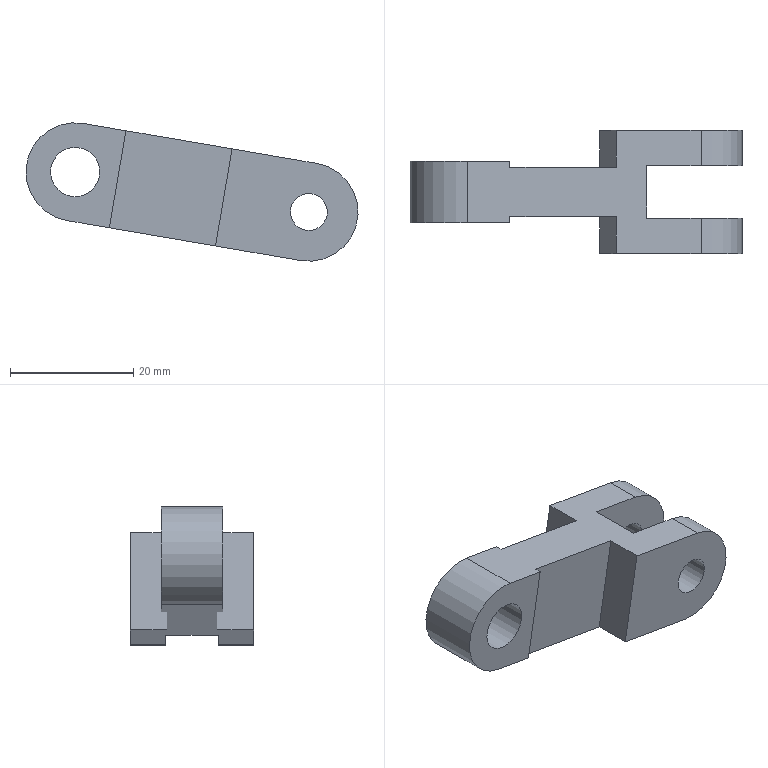Component | NX | CLHKJG_12_CONNECTING_ROD | 1 solid | 21 faces | volume 7950 mm3 | plane 15 | cylinder 6 | commonest cylinder face diameters 16 x3 6 x2 8 x1